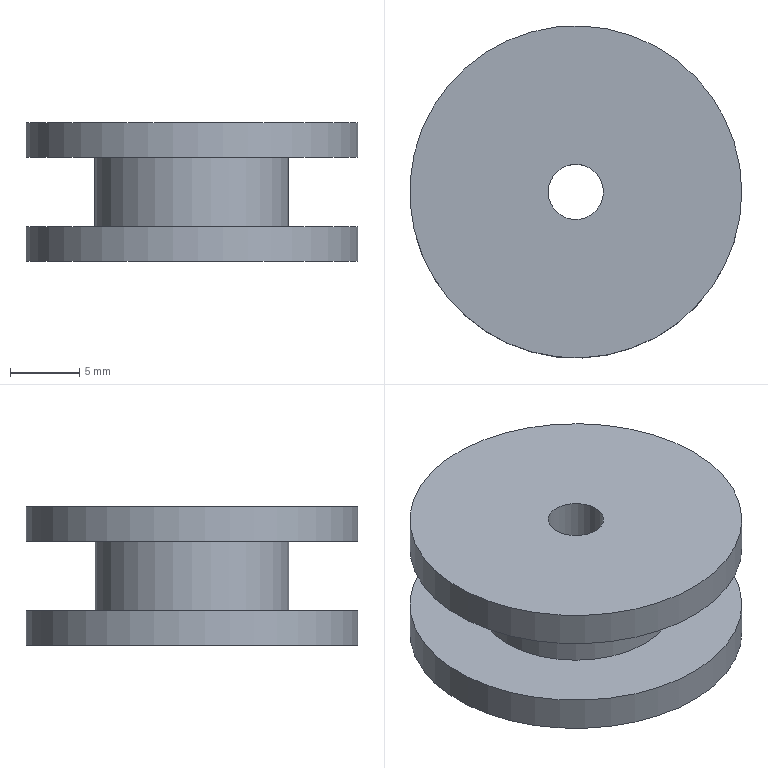Component | NX | PISTON | 1 solid | 10 faces | box 24 x 24 x 10 mm | volume 2827 mm3 | plane 5 | cylinder 5 | commonest cylinder face diameters 24 x2 14 x1 6 x1 4 x1
STEP:
#1=CARTESIAN_POINT('',(0.,0.,0.));
#2=DIRECTION('',(0.,0.,1.));
#3=DIRECTION('',(1.,0.,0.));
#4=AXIS2_PLACEMENT_3D('',#1,#2,#3);
#5=CARTESIAN_POINT('',(3.,-10.,150.121));
#6=VERTEX_POINT('',#5);
#7=CARTESIAN_POINT('',(-0.,-10.,150.121));
#8=DIRECTION('',(0.,0.,1.));
#9=DIRECTION('',(1.,0.,0.));
#10=AXIS2_PLACEMENT_3D('',#7,#8,#9);
#11=CIRCLE('',#10,3.);
#12=CARTESIAN_POINT('',(-0.,-22.,150.121));
#13=DIRECTION('',(0.,0.,-1.));
#14=DIRECTION('',(-1.,0.,0.));
#15=AXIS2_PLACEMENT_3D('',#12,#13,#14);
#16=PLANE('',#15);
#17=CARTESIAN_POINT('',(-3.,12.));
#18=CARTESIAN_POINT('',(-3.,17.196));
#19=CARTESIAN_POINT('',(1.5,14.598));
#20=CARTESIAN_POINT('',(6.,12.));
#21=CARTESIAN_POINT('',(1.5,9.402));
#22=CARTESIAN_POINT('',(-3.,6.804));
#23=CARTESIAN_POINT('',(-3.,12.));
#24=(BOUNDED_CURVE()B_SPLINE_CURVE(2,(#17,#18,#19,#20,#21,#22,#23),.UNSPECIFIED.,.T.,.F.)B_SPLINE_CURVE_WITH_KNOTS((1,2,2,2,2,1),(-2.094,0.,2.094,4.189,6.283,8.378),.UNSPECIFIED.)CURVE()GEOMETRIC_REPRESENTATION_ITEM()RATIONAL_B_SPLINE_CURVE((1.,0.5,1.,0.5,1.,0.5,1.))REPRESENTATION_ITEM(''));
#25=(GEOMETRIC_REPRESENTATION_CONTEXT(2)PARAMETRIC_REPRESENTATION_CONTEXT()REPRESENTATION_CONTEXT('',''));
#26=DEFINITIONAL_REPRESENTATION('',(#24),#25);
#27=PCURVE('',#16,#26);
#28=CARTESIAN_POINT('',(-0.,-10.,155.121));
#29=DIRECTION('',(0.,0.,-1.));
#30=DIRECTION('',(-1.,0.,0.));
#31=AXIS2_PLACEMENT_3D('',#28,#29,#30);
#32=CYLINDRICAL_SURFACE('',#31,3.);
#33=CARTESIAN_POINT('',(9.425,5.));
#34=DIRECTION('',(-1.,0.));
#35=VECTOR('',#34,1.);
#36=LINE('',#33,#35);
#37=(GEOMETRIC_REPRESENTATION_CONTEXT(2)PARAMETRIC_REPRESENTATION_CONTEXT()REPRESENTATION_CONTEXT('',''));
#38=DEFINITIONAL_REPRESENTATION('',(#36),#37);
#39=PCURVE('',#32,#38);
#40=SURFACE_CURVE('',#11,(#27,#39),.PCURVE_S1.);
#41=EDGE_CURVE('',#6,#6,#40,.T.);
#42=ORIENTED_EDGE('',*,*,#41,.T.);
#43=EDGE_LOOP('',(#42));
#44=FACE_BOUND('',#43,.T.);
#45=CARTESIAN_POINT('',(12.,-10.,150.121));
#46=VERTEX_POINT('',#45);
#47=CARTESIAN_POINT('',(-0.,-10.,150.121));
#48=DIRECTION('',(0.,0.,1.));
#49=DIRECTION('',(1.,0.,0.));
#50=AXIS2_PLACEMENT_3D('',#47,#48,#49);
#51=CIRCLE('',#50,12.);
#52=CARTESIAN_POINT('',(-12.,12.));
#53=CARTESIAN_POINT('',(-12.,32.785));
#54=CARTESIAN_POINT('',(6.,22.392));
#55=CARTESIAN_POINT('',(24.,12.));
#56=CARTESIAN_POINT('',(6.,1.608));
#57=CARTESIAN_POINT('',(-12.,-8.785));
#58=CARTESIAN_POINT('',(-12.,12.));
#59=(BOUNDED_CURVE()B_SPLINE_CURVE(2,(#52,#53,#54,#55,#56,#57,#58),.UNSPECIFIED.,.T.,.F.)B_SPLINE_CURVE_WITH_KNOTS((1,2,2,2,2,1),(-2.094,0.,2.094,4.189,6.283,8.378),.UNSPECIFIED.)CURVE()GEOMETRIC_REPRESENTATION_ITEM()RATIONAL_B_SPLINE_CURVE((1.,0.5,1.,0.5,1.,0.5,1.))REPRESENTATION_ITEM(''));
#60=(GEOMETRIC_REPRESENTATION_CONTEXT(2)PARAMETRIC_REPRESENTATION_CONTEXT()REPRESENTATION_CONTEXT('',''));
#61=DEFINITIONAL_REPRESENTATION('',(#59),#60);
#62=PCURVE('',#16,#61);
#63=CARTESIAN_POINT('',(-0.,-10.,150.121));
#64=DIRECTION('',(0.,0.,1.));
#65=DIRECTION('',(1.,0.,0.));
#66=AXIS2_PLACEMENT_3D('',#63,#64,#65);
#67=CYLINDRICAL_SURFACE('',#66,12.);
#68=CARTESIAN_POINT('',(0.,0.));
#69=DIRECTION('',(1.,0.));
#70=VECTOR('',#69,1.);
#71=LINE('',#68,#70);
#72=(GEOMETRIC_REPRESENTATION_CONTEXT(2)PARAMETRIC_REPRESENTATION_CONTEXT()REPRESENTATION_CONTEXT('',''));
#73=DEFINITIONAL_REPRESENTATION('',(#71),#72);
#74=PCURVE('',#67,#73);
#75=SURFACE_CURVE('',#51,(#62,#74),.PCURVE_S1.);
#76=EDGE_CURVE('',#46,#46,#75,.T.);
#77=ORIENTED_EDGE('',*,*,#76,.F.);
#78=EDGE_LOOP('',(#77));
#79=FACE_BOUND('',#78,.T.);
#80=ADVANCED_FACE('',(#44,#79),#16,.T.);
#81=ORIENTED_EDGE('',*,*,#76,.T.);
#82=CARTESIAN_POINT('',(12.,-10.,152.621));
#83=VERTEX_POINT('',#82);
#84=CARTESIAN_POINT('',(12.,-10.,150.121));
#85=CARTESIAN_POINT('',(12.,-10.,152.621));
#86=B_SPLINE_CURVE_WITH_KNOTS('',1,(#84,#85),.UNSPECIFIED.,.F.,.F.,(2,2),(0.,2.5),.PIECEWISE_BEZIER_KNOTS.);
#87=CARTESIAN_POINT('',(6.283,0.));
#88=DIRECTION('',(0.,1.));
#89=VECTOR('',#88,1.);
#90=LINE('',#87,#89);
#91=(GEOMETRIC_REPRESENTATION_CONTEXT(2)PARAMETRIC_REPRESENTATION_CONTEXT()REPRESENTATION_CONTEXT('',''));
#92=DEFINITIONAL_REPRESENTATION('',(#90),#91);
#93=PCURVE('',#67,#92);
#94=CARTESIAN_POINT('',(0.,0.));
#95=DIRECTION('',(0.,1.));
#96=VECTOR('',#95,1.);
#97=LINE('',#94,#96);
#98=(GEOMETRIC_REPRESENTATION_CONTEXT(2)PARAMETRIC_REPRESENTATION_CONTEXT()REPRESENTATION_CONTEXT('',''));
#99=DEFINITIONAL_REPRESENTATION('',(#97),#98);
#100=PCURVE('',#67,#99);
#101=SEAM_CURVE('',#86,(#93,#100),.PCURVE_S1.);
#102=EDGE_CURVE('',#46,#83,#101,.T.);
#103=ORIENTED_EDGE('',*,*,#102,.T.);
#104=CARTESIAN_POINT('',(-0.,-10.,152.621));
#105=DIRECTION('',(0.,0.,1.));
#106=DIRECTION('',(1.,0.,0.));
#107=AXIS2_PLACEMENT_3D('',#104,#105,#106);
#108=CIRCLE('',#107,12.);
#109=CARTESIAN_POINT('',(0.,2.5));
#110=DIRECTION('',(1.,0.));
#111=VECTOR('',#110,1.);
#112=LINE('',#109,#111);
#113=(GEOMETRIC_REPRESENTATION_CONTEXT(2)PARAMETRIC_REPRESENTATION_CONTEXT()REPRESENTATION_CONTEXT('',''));
#114=DEFINITIONAL_REPRESENTATION('',(#112),#113);
#115=PCURVE('',#67,#114);
#116=CARTESIAN_POINT('',(-0.,-17.,152.621));
#117=DIRECTION('',(0.,0.,1.));
#118=DIRECTION('',(1.,0.,0.));
#119=AXIS2_PLACEMENT_3D('',#116,#117,#118);
#120=PLANE('',#119);
#121=CARTESIAN_POINT('',(0.,7.));
#122=DIRECTION('',(1.,0.));
#123=AXIS2_PLACEMENT_2D('',#121,#122);
#124=CIRCLE('',#123,12.);
#125=(GEOMETRIC_REPRESENTATION_CONTEXT(2)PARAMETRIC_REPRESENTATION_CONTEXT()REPRESENTATION_CONTEXT('',''));
#126=DEFINITIONAL_REPRESENTATION('',(#124),#125);
#127=PCURVE('',#120,#126);
#128=SURFACE_CURVE('',#108,(#115,#127),.PCURVE_S1.);
#129=EDGE_CURVE('',#83,#83,#128,.T.);
#130=ORIENTED_EDGE('',*,*,#129,.F.);
#131=ORIENTED_EDGE('',*,*,#102,.F.);
#132=EDGE_LOOP('',(#81,#103,#130,#131));
#133=FACE_BOUND('',#132,.T.);
#134=ADVANCED_FACE('',(#133),#67,.T.);
#135=ORIENTED_EDGE('',*,*,#129,.T.);
#136=EDGE_LOOP('',(#135));
#137=FACE_BOUND('',#136,.T.);
#138=CARTESIAN_POINT('',(7.,-10.,152.621));
#139=VERTEX_POINT('',#138);
#140=CARTESIAN_POINT('',(-0.,-10.,152.621));
#141=DIRECTION('',(0.,0.,1.));
#142=DIRECTION('',(1.,0.,0.));
#143=AXIS2_PLACEMENT_3D('',#140,#141,#142);
#144=CIRCLE('',#143,7.);
#145=CARTESIAN_POINT('',(0.,7.));
#146=DIRECTION('',(1.,0.));
#147=AXIS2_PLACEMENT_2D('',#145,#146);
#148=CIRCLE('',#147,7.);
#149=(GEOMETRIC_REPRESENTATION_CONTEXT(2)PARAMETRIC_REPRESENTATION_CONTEXT()REPRESENTATION_CONTEXT('',''));
#150=DEFINITIONAL_REPRESENTATION('',(#148),#149);
#151=PCURVE('',#120,#150);
#152=CARTESIAN_POINT('',(-0.,-10.,150.121));
#153=DIRECTION('',(0.,0.,1.));
#154=DIRECTION('',(1.,0.,0.));
#155=AXIS2_PLACEMENT_3D('',#152,#153,#154);
#156=CYLINDRICAL_SURFACE('',#155,7.);
#157=CARTESIAN_POINT('',(0.,2.5));
#158=DIRECTION('',(1.,0.));
#159=VECTOR('',#158,1.);
#160=LINE('',#157,#159);
#161=(GEOMETRIC_REPRESENTATION_CONTEXT(2)PARAMETRIC_REPRESENTATION_CONTEXT()REPRESENTATION_CONTEXT('',''));
#162=DEFINITIONAL_REPRESENTATION('',(#160),#161);
#163=PCURVE('',#156,#162);
#164=SURFACE_CURVE('',#144,(#151,#163),.PCURVE_S1.);
#165=EDGE_CURVE('',#139,#139,#164,.T.);
#166=ORIENTED_EDGE('',*,*,#165,.F.);
#167=EDGE_LOOP('',(#166));
#168=FACE_BOUND('',#167,.T.);
#169=ADVANCED_FACE('',(#137,#168),#120,.T.);
#170=ORIENTED_EDGE('',*,*,#165,.T.);
#171=CARTESIAN_POINT('',(7.,-10.,157.621));
#172=VERTEX_POINT('',#171);
#173=CARTESIAN_POINT('',(7.,-10.,152.621));
#174=CARTESIAN_POINT('',(7.,-10.,157.621));
#175=B_SPLINE_CURVE_WITH_KNOTS('',1,(#173,#174),.UNSPECIFIED.,.F.,.F.,(2,2),(2.5,7.5),.PIECEWISE_BEZIER_KNOTS.);
#176=CARTESIAN_POINT('',(6.283,0.));
#177=DIRECTION('',(0.,1.));
#178=VECTOR('',#177,1.);
#179=LINE('',#176,#178);
#180=(GEOMETRIC_REPRESENTATION_CONTEXT(2)PARAMETRIC_REPRESENTATION_CONTEXT()REPRESENTATION_CONTEXT('',''));
#181=DEFINITIONAL_REPRESENTATION('',(#179),#180);
#182=PCURVE('',#156,#181);
#183=CARTESIAN_POINT('',(0.,0.));
#184=DIRECTION('',(0.,1.));
#185=VECTOR('',#184,1.);
#186=LINE('',#183,#185);
#187=(GEOMETRIC_REPRESENTATION_CONTEXT(2)PARAMETRIC_REPRESENTATION_CONTEXT()REPRESENTATION_CONTEXT('',''));
#188=DEFINITIONAL_REPRESENTATION('',(#186),#187);
#189=PCURVE('',#156,#188);
#190=SEAM_CURVE('',#175,(#182,#189),.PCURVE_S1.);
#191=EDGE_CURVE('',#139,#172,#190,.T.);
#192=ORIENTED_EDGE('',*,*,#191,.T.);
#193=CARTESIAN_POINT('',(-0.,-10.,157.621));
#194=DIRECTION('',(0.,0.,1.));
#195=DIRECTION('',(1.,0.,0.));
#196=AXIS2_PLACEMENT_3D('',#193,#194,#195);
#197=CIRCLE('',#196,7.);
#198=CARTESIAN_POINT('',(0.,7.5));
#199=DIRECTION('',(1.,0.));
#200=VECTOR('',#199,1.);
#201=LINE('',#198,#200);
#202=(GEOMETRIC_REPRESENTATION_CONTEXT(2)PARAMETRIC_REPRESENTATION_CONTEXT()REPRESENTATION_CONTEXT('',''));
#203=DEFINITIONAL_REPRESENTATION('',(#201),#202);
#204=PCURVE('',#156,#203);
#205=CARTESIAN_POINT('',(-0.,-22.,157.621));
#206=DIRECTION('',(0.,0.,-1.));
#207=DIRECTION('',(-1.,0.,0.));
#208=AXIS2_PLACEMENT_3D('',#205,#206,#207);
#209=PLANE('',#208);
#210=CARTESIAN_POINT('',(-7.,12.));
#211=CARTESIAN_POINT('',(-7.,24.124));
#212=CARTESIAN_POINT('',(3.5,18.062));
#213=CARTESIAN_POINT('',(14.,12.));
#214=CARTESIAN_POINT('',(3.5,5.938));
#215=CARTESIAN_POINT('',(-7.,-0.1244));
#216=CARTESIAN_POINT('',(-7.,12.));
#217=(BOUNDED_CURVE()B_SPLINE_CURVE(2,(#210,#211,#212,#213,#214,#215,#216),.UNSPECIFIED.,.T.,.F.)B_SPLINE_CURVE_WITH_KNOTS((1,2,2,2,2,1),(-2.094,0.,2.094,4.189,6.283,8.378),.UNSPECIFIED.)CURVE()GEOMETRIC_REPRESENTATION_ITEM()RATIONAL_B_SPLINE_CURVE((1.,0.5,1.,0.5,1.,0.5,1.))REPRESENTATION_ITEM(''));
#218=(GEOMETRIC_REPRESENTATION_CONTEXT(2)PARAMETRIC_REPRESENTATION_CONTEXT()REPRESENTATION_CONTEXT('',''));
#219=DEFINITIONAL_REPRESENTATION('',(#217),#218);
#220=PCURVE('',#209,#219);
#221=SURFACE_CURVE('',#197,(#204,#220),.PCURVE_S1.);
#222=EDGE_CURVE('',#172,#172,#221,.T.);
#223=ORIENTED_EDGE('',*,*,#222,.F.);
#224=ORIENTED_EDGE('',*,*,#191,.F.);
#225=EDGE_LOOP('',(#170,#192,#223,#224));
#226=FACE_BOUND('',#225,.T.);
#227=ADVANCED_FACE('',(#226),#156,.T.);
#228=ORIENTED_EDGE('',*,*,#222,.T.);
#229=EDGE_LOOP('',(#228));
#230=FACE_BOUND('',#229,.T.);
#231=CARTESIAN_POINT('',(12.,-10.,157.621));
#232=VERTEX_POINT('',#231);
#233=CARTESIAN_POINT('',(-0.,-10.,157.621));
#234=DIRECTION('',(0.,0.,1.));
#235=DIRECTION('',(1.,0.,0.));
#236=AXIS2_PLACEMENT_3D('',#233,#234,#235);
#237=CIRCLE('',#236,12.);
#238=CARTESIAN_POINT('',(-12.,12.));
#239=CARTESIAN_POINT('',(-12.,32.785));
#240=CARTESIAN_POINT('',(6.,22.392));
#241=CARTESIAN_POINT('',(24.,12.));
#242=CARTESIAN_POINT('',(6.,1.608));
#243=CARTESIAN_POINT('',(-12.,-8.785));
#244=CARTESIAN_POINT('',(-12.,12.));
#245=(BOUNDED_CURVE()B_SPLINE_CURVE(2,(#238,#239,#240,#241,#242,#243,#244),.UNSPECIFIED.,.T.,.F.)B_SPLINE_CURVE_WITH_KNOTS((1,2,2,2,2,1),(-2.094,0.,2.094,4.189,6.283,8.378),.UNSPECIFIED.)CURVE()GEOMETRIC_REPRESENTATION_ITEM()RATIONAL_B_SPLINE_CURVE((1.,0.5,1.,0.5,1.,0.5,1.))REPRESENTATION_ITEM(''));
#246=(GEOMETRIC_REPRESENTATION_CONTEXT(2)PARAMETRIC_REPRESENTATION_CONTEXT()REPRESENTATION_CONTEXT('',''));
#247=DEFINITIONAL_REPRESENTATION('',(#245),#246);
#248=PCURVE('',#209,#247);
#249=CARTESIAN_POINT('',(-0.,-10.,150.121));
#250=DIRECTION('',(0.,0.,1.));
#251=DIRECTION('',(1.,0.,0.));
#252=AXIS2_PLACEMENT_3D('',#249,#250,#251);
#253=CYLINDRICAL_SURFACE('',#252,12.);
#254=CARTESIAN_POINT('',(0.,7.5));
#255=DIRECTION('',(1.,0.));
#256=VECTOR('',#255,1.);
#257=LINE('',#254,#256);
#258=(GEOMETRIC_REPRESENTATION_CONTEXT(2)PARAMETRIC_REPRESENTATION_CONTEXT()REPRESENTATION_CONTEXT('',''));
#259=DEFINITIONAL_REPRESENTATION('',(#257),#258);
#260=PCURVE('',#253,#259);
#261=SURFACE_CURVE('',#237,(#248,#260),.PCURVE_S1.);
#262=EDGE_CURVE('',#232,#232,#261,.T.);
#263=ORIENTED_EDGE('',*,*,#262,.F.);
#264=EDGE_LOOP('',(#263));
#265=FACE_BOUND('',#264,.T.);
#266=ADVANCED_FACE('',(#230,#265),#209,.T.);
#267=ORIENTED_EDGE('',*,*,#262,.T.);
#268=CARTESIAN_POINT('',(12.,-10.,160.121));
#269=VERTEX_POINT('',#268);
#270=CARTESIAN_POINT('',(12.,-10.,157.621));
#271=CARTESIAN_POINT('',(12.,-10.,160.121));
#272=B_SPLINE_CURVE_WITH_KNOTS('',1,(#270,#271),.UNSPECIFIED.,.F.,.F.,(2,2),(7.5,10.),.PIECEWISE_BEZIER_KNOTS.);
#273=CARTESIAN_POINT('',(6.283,0.));
#274=DIRECTION('',(0.,1.));
#275=VECTOR('',#274,1.);
#276=LINE('',#273,#275);
#277=(GEOMETRIC_REPRESENTATION_CONTEXT(2)PARAMETRIC_REPRESENTATION_CONTEXT()REPRESENTATION_CONTEXT('',''));
#278=DEFINITIONAL_REPRESENTATION('',(#276),#277);
#279=PCURVE('',#253,#278);
#280=CARTESIAN_POINT('',(0.,0.));
#281=DIRECTION('',(0.,1.));
#282=VECTOR('',#281,1.);
#283=LINE('',#280,#282);
#284=(GEOMETRIC_REPRESENTATION_CONTEXT(2)PARAMETRIC_REPRESENTATION_CONTEXT()REPRESENTATION_CONTEXT('',''));
#285=DEFINITIONAL_REPRESENTATION('',(#283),#284);
#286=PCURVE('',#253,#285);
#287=SEAM_CURVE('',#272,(#279,#286),.PCURVE_S1.);
#288=EDGE_CURVE('',#232,#269,#287,.T.);
#289=ORIENTED_EDGE('',*,*,#288,.T.);
#290=CARTESIAN_POINT('',(-0.,-10.,160.121));
#291=DIRECTION('',(0.,0.,1.));
#292=DIRECTION('',(1.,0.,0.));
#293=AXIS2_PLACEMENT_3D('',#290,#291,#292);
#294=CIRCLE('',#293,12.);
#295=CARTESIAN_POINT('',(0.,10.));
#296=DIRECTION('',(1.,0.));
#297=VECTOR('',#296,1.);
#298=LINE('',#295,#297);
#299=(GEOMETRIC_REPRESENTATION_CONTEXT(2)PARAMETRIC_REPRESENTATION_CONTEXT()REPRESENTATION_CONTEXT('',''));
#300=DEFINITIONAL_REPRESENTATION('',(#298),#299);
#301=PCURVE('',#253,#300);
#302=CARTESIAN_POINT('',(-0.,-10.,160.121));
#303=DIRECTION('',(0.,0.,1.));
#304=DIRECTION('',(1.,0.,0.));
#305=AXIS2_PLACEMENT_3D('',#302,#303,#304);
#306=PLANE('',#305);
#307=CARTESIAN_POINT('',(0.,0.));
#308=DIRECTION('',(1.,0.));
#309=AXIS2_PLACEMENT_2D('',#307,#308);
#310=CIRCLE('',#309,12.);
#311=(GEOMETRIC_REPRESENTATION_CONTEXT(2)PARAMETRIC_REPRESENTATION_CONTEXT()REPRESENTATION_CONTEXT('',''));
#312=DEFINITIONAL_REPRESENTATION('',(#310),#311);
#313=PCURVE('',#306,#312);
#314=SURFACE_CURVE('',#294,(#301,#313),.PCURVE_S1.);
#315=EDGE_CURVE('',#269,#269,#314,.T.);
#316=ORIENTED_EDGE('',*,*,#315,.F.);
#317=ORIENTED_EDGE('',*,*,#288,.F.);
#318=EDGE_LOOP('',(#267,#289,#316,#317));
#319=FACE_BOUND('',#318,.T.);
#320=ADVANCED_FACE('',(#319),#253,.T.);
#321=CARTESIAN_POINT('',(2.,-10.,160.121));
#322=VERTEX_POINT('',#321);
#323=CARTESIAN_POINT('',(-0.,-10.,160.121));
#324=DIRECTION('',(0.,0.,-1.));
#325=DIRECTION('',(1.,0.,0.));
#326=AXIS2_PLACEMENT_3D('',#323,#324,#325);
#327=CIRCLE('',#326,2.);
#328=CARTESIAN_POINT('',(2.,0.));
#329=CARTESIAN_POINT('',(2.,-3.464));
#330=CARTESIAN_POINT('',(-1.,-1.732));
#331=CARTESIAN_POINT('',(-4.,-0.));
#332=CARTESIAN_POINT('',(-1.,1.732));
#333=CARTESIAN_POINT('',(2.,3.464));
#334=CARTESIAN_POINT('',(2.,0.));
#335=(BOUNDED_CURVE()B_SPLINE_CURVE(2,(#328,#329,#330,#331,#332,#333,#334),.UNSPECIFIED.,.T.,.F.)B_SPLINE_CURVE_WITH_KNOTS((1,2,2,2,2,1),(-2.094,0.,2.094,4.189,6.283,8.378),.UNSPECIFIED.)CURVE()GEOMETRIC_REPRESENTATION_ITEM()RATIONAL_B_SPLINE_CURVE((1.,0.5,1.,0.5,1.,0.5,1.))REPRESENTATION_ITEM(''));
#336=(GEOMETRIC_REPRESENTATION_CONTEXT(2)PARAMETRIC_REPRESENTATION_CONTEXT()REPRESENTATION_CONTEXT('',''));
#337=DEFINITIONAL_REPRESENTATION('',(#335),#336);
#338=PCURVE('',#306,#337);
#339=CARTESIAN_POINT('',(-0.,-10.,165.121));
#340=DIRECTION('',(0.,0.,-1.));
#341=DIRECTION('',(-1.,0.,0.));
#342=AXIS2_PLACEMENT_3D('',#339,#340,#341);
#343=CYLINDRICAL_SURFACE('',#342,2.);
#344=CARTESIAN_POINT('',(3.142,5.));
#345=DIRECTION('',(1.,0.));
#346=VECTOR('',#345,1.);
#347=LINE('',#344,#346);
#348=(GEOMETRIC_REPRESENTATION_CONTEXT(2)PARAMETRIC_REPRESENTATION_CONTEXT()REPRESENTATION_CONTEXT('',''));
#349=DEFINITIONAL_REPRESENTATION('',(#347),#348);
#350=PCURVE('',#343,#349);
#351=SURFACE_CURVE('',#327,(#338,#350),.PCURVE_S1.);
#352=EDGE_CURVE('',#322,#322,#351,.T.);
#353=ORIENTED_EDGE('',*,*,#352,.T.);
#354=EDGE_LOOP('',(#353));
#355=FACE_BOUND('',#354,.T.);
#356=ORIENTED_EDGE('',*,*,#315,.T.);
#357=EDGE_LOOP('',(#356));
#358=FACE_BOUND('',#357,.T.);
#359=ADVANCED_FACE('',(#355,#358),#306,.T.);
#360=CARTESIAN_POINT('',(3.,-10.,155.121));
#361=VERTEX_POINT('',#360);
#362=CARTESIAN_POINT('',(-0.,-10.,155.121));
#363=DIRECTION('',(0.,0.,-1.));
#364=DIRECTION('',(1.,0.,0.));
#365=AXIS2_PLACEMENT_3D('',#362,#363,#364);
#366=CIRCLE('',#365,3.);
#367=CARTESIAN_POINT('',(3.142,0.));
#368=DIRECTION('',(1.,0.));
#369=VECTOR('',#368,1.);
#370=LINE('',#367,#369);
#371=(GEOMETRIC_REPRESENTATION_CONTEXT(2)PARAMETRIC_REPRESENTATION_CONTEXT()REPRESENTATION_CONTEXT('',''));
#372=DEFINITIONAL_REPRESENTATION('',(#370),#371);
#373=PCURVE('',#32,#372);
#374=CARTESIAN_POINT('',(-0.,-10.,155.121));
#375=DIRECTION('',(0.,0.,1.));
#376=DIRECTION('',(1.,0.,0.));
#377=AXIS2_PLACEMENT_3D('',#374,#375,#376);
#378=PLANE('',#377);
#379=CARTESIAN_POINT('',(3.,0.));
#380=CARTESIAN_POINT('',(3.,-5.196));
#381=CARTESIAN_POINT('',(-1.5,-2.598));
#382=CARTESIAN_POINT('',(-6.,-0.));
#383=CARTESIAN_POINT('',(-1.5,2.598));
#384=CARTESIAN_POINT('',(3.,5.196));
#385=CARTESIAN_POINT('',(3.,0.));
#386=(BOUNDED_CURVE()B_SPLINE_CURVE(2,(#379,#380,#381,#382,#383,#384,#385),.UNSPECIFIED.,.T.,.F.)B_SPLINE_CURVE_WITH_KNOTS((1,2,2,2,2,1),(-2.094,0.,2.094,4.189,6.283,8.378),.UNSPECIFIED.)CURVE()GEOMETRIC_REPRESENTATION_ITEM()RATIONAL_B_SPLINE_CURVE((1.,0.5,1.,0.5,1.,0.5,1.))REPRESENTATION_ITEM(''));
#387=(GEOMETRIC_REPRESENTATION_CONTEXT(2)PARAMETRIC_REPRESENTATION_CONTEXT()REPRESENTATION_CONTEXT('',''));
#388=DEFINITIONAL_REPRESENTATION('',(#386),#387);
#389=PCURVE('',#378,#388);
#390=SURFACE_CURVE('',#366,(#373,#389),.PCURVE_S1.);
#391=EDGE_CURVE('',#361,#361,#390,.T.);
#392=ORIENTED_EDGE('',*,*,#391,.T.);
#393=CARTESIAN_POINT('',(3.,-10.,155.121));
#394=CARTESIAN_POINT('',(3.,-10.,150.121));
#395=B_SPLINE_CURVE_WITH_KNOTS('',1,(#393,#394),.UNSPECIFIED.,.F.,.F.,(2,2),(0.,5.),.PIECEWISE_BEZIER_KNOTS.);
#396=CARTESIAN_POINT('',(9.425,0.));
#397=DIRECTION('',(0.,1.));
#398=VECTOR('',#397,1.);
#399=LINE('',#396,#398);
#400=(GEOMETRIC_REPRESENTATION_CONTEXT(2)PARAMETRIC_REPRESENTATION_CONTEXT()REPRESENTATION_CONTEXT('',''));
#401=DEFINITIONAL_REPRESENTATION('',(#399),#400);
#402=PCURVE('',#32,#401);
#403=CARTESIAN_POINT('',(3.142,0.));
#404=DIRECTION('',(0.,1.));
#405=VECTOR('',#404,1.);
#406=LINE('',#403,#405);
#407=(GEOMETRIC_REPRESENTATION_CONTEXT(2)PARAMETRIC_REPRESENTATION_CONTEXT()REPRESENTATION_CONTEXT('',''));
#408=DEFINITIONAL_REPRESENTATION('',(#406),#407);
#409=PCURVE('',#32,#408);
#410=SEAM_CURVE('',#395,(#402,#409),.PCURVE_S1.);
#411=EDGE_CURVE('',#361,#6,#410,.T.);
#412=ORIENTED_EDGE('',*,*,#411,.T.);
#413=ORIENTED_EDGE('',*,*,#41,.T.);
#414=ORIENTED_EDGE('',*,*,#411,.F.);
#415=EDGE_LOOP('',(#392,#412,#413,#414));
#416=FACE_BOUND('',#415,.F.);
#417=ADVANCED_FACE('',(#416),#32,.F.);
#418=CARTESIAN_POINT('',(2.,-10.,155.121));
#419=VERTEX_POINT('',#418);
#420=CARTESIAN_POINT('',(-0.,-10.,155.121));
#421=DIRECTION('',(0.,0.,1.));
#422=DIRECTION('',(1.,0.,0.));
#423=AXIS2_PLACEMENT_3D('',#420,#421,#422);
#424=CIRCLE('',#423,2.);
#425=CARTESIAN_POINT('',(0.,0.));
#426=DIRECTION('',(1.,0.));
#427=AXIS2_PLACEMENT_2D('',#425,#426);
#428=CIRCLE('',#427,2.);
#429=(GEOMETRIC_REPRESENTATION_CONTEXT(2)PARAMETRIC_REPRESENTATION_CONTEXT()REPRESENTATION_CONTEXT('',''));
#430=DEFINITIONAL_REPRESENTATION('',(#428),#429);
#431=PCURVE('',#378,#430);
#432=CARTESIAN_POINT('',(9.425,10.));
#433=DIRECTION('',(-1.,0.));
#434=VECTOR('',#433,1.);
#435=LINE('',#432,#434);
#436=(GEOMETRIC_REPRESENTATION_CONTEXT(2)PARAMETRIC_REPRESENTATION_CONTEXT()REPRESENTATION_CONTEXT('',''));
#437=DEFINITIONAL_REPRESENTATION('',(#435),#436);
#438=PCURVE('',#343,#437);
#439=SURFACE_CURVE('',#424,(#431,#438),.PCURVE_S1.);
#440=EDGE_CURVE('',#419,#419,#439,.T.);
#441=ORIENTED_EDGE('',*,*,#440,.T.);
#442=EDGE_LOOP('',(#441));
#443=FACE_BOUND('',#442,.T.);
#444=ORIENTED_EDGE('',*,*,#391,.T.);
#445=EDGE_LOOP('',(#444));
#446=FACE_BOUND('',#445,.T.);
#447=ADVANCED_FACE('',(#443,#446),#378,.F.);
#448=ORIENTED_EDGE('',*,*,#352,.T.);
#449=CARTESIAN_POINT('',(2.,-10.,160.121));
#450=CARTESIAN_POINT('',(2.,-10.,155.121));
#451=B_SPLINE_CURVE_WITH_KNOTS('',1,(#449,#450),.UNSPECIFIED.,.F.,.F.,(2,2),(5.,10.),.PIECEWISE_BEZIER_KNOTS.);
#452=CARTESIAN_POINT('',(9.425,0.));
#453=DIRECTION('',(0.,1.));
#454=VECTOR('',#453,1.);
#455=LINE('',#452,#454);
#456=(GEOMETRIC_REPRESENTATION_CONTEXT(2)PARAMETRIC_REPRESENTATION_CONTEXT()REPRESENTATION_CONTEXT('',''));
#457=DEFINITIONAL_REPRESENTATION('',(#455),#456);
#458=PCURVE('',#343,#457);
#459=CARTESIAN_POINT('',(3.142,0.));
#460=DIRECTION('',(0.,1.));
#461=VECTOR('',#460,1.);
#462=LINE('',#459,#461);
#463=(GEOMETRIC_REPRESENTATION_CONTEXT(2)PARAMETRIC_REPRESENTATION_CONTEXT()REPRESENTATION_CONTEXT('',''));
#464=DEFINITIONAL_REPRESENTATION('',(#462),#463);
#465=PCURVE('',#343,#464);
#466=SEAM_CURVE('',#451,(#458,#465),.PCURVE_S1.);
#467=EDGE_CURVE('',#322,#419,#466,.T.);
#468=ORIENTED_EDGE('',*,*,#467,.T.);
#469=ORIENTED_EDGE('',*,*,#440,.T.);
#470=ORIENTED_EDGE('',*,*,#467,.F.);
#471=EDGE_LOOP('',(#448,#468,#469,#470));
#472=FACE_BOUND('',#471,.F.);
#473=ADVANCED_FACE('',(#472),#343,.F.);
#474=CLOSED_SHELL('',(#80,#134,#169,#227,#266,#320,#359,#417,#447,#473));
#475=MANIFOLD_SOLID_BREP('',#474);
#476=(LENGTH_UNIT()NAMED_UNIT(*)SI_UNIT(.MILLI.,.METRE.));
#477=UNCERTAINTY_MEASURE_WITH_UNIT(LENGTH_MEASURE(0.00001),#476,'','');
#478=(NAMED_UNIT(*)PLANE_ANGLE_UNIT()SI_UNIT($,.RADIAN.));
#479=(NAMED_UNIT(*)SI_UNIT($,.STERADIAN.)SOLID_ANGLE_UNIT());
#480=(GEOMETRIC_REPRESENTATION_CONTEXT(3)GLOBAL_UNCERTAINTY_ASSIGNED_CONTEXT((#477))GLOBAL_UNIT_ASSIGNED_CONTEXT((#476,#478,#479))REPRESENTATION_CONTEXT('',''));
#481=ADVANCED_BREP_SHAPE_REPRESENTATION('',(#4,#475),#480);